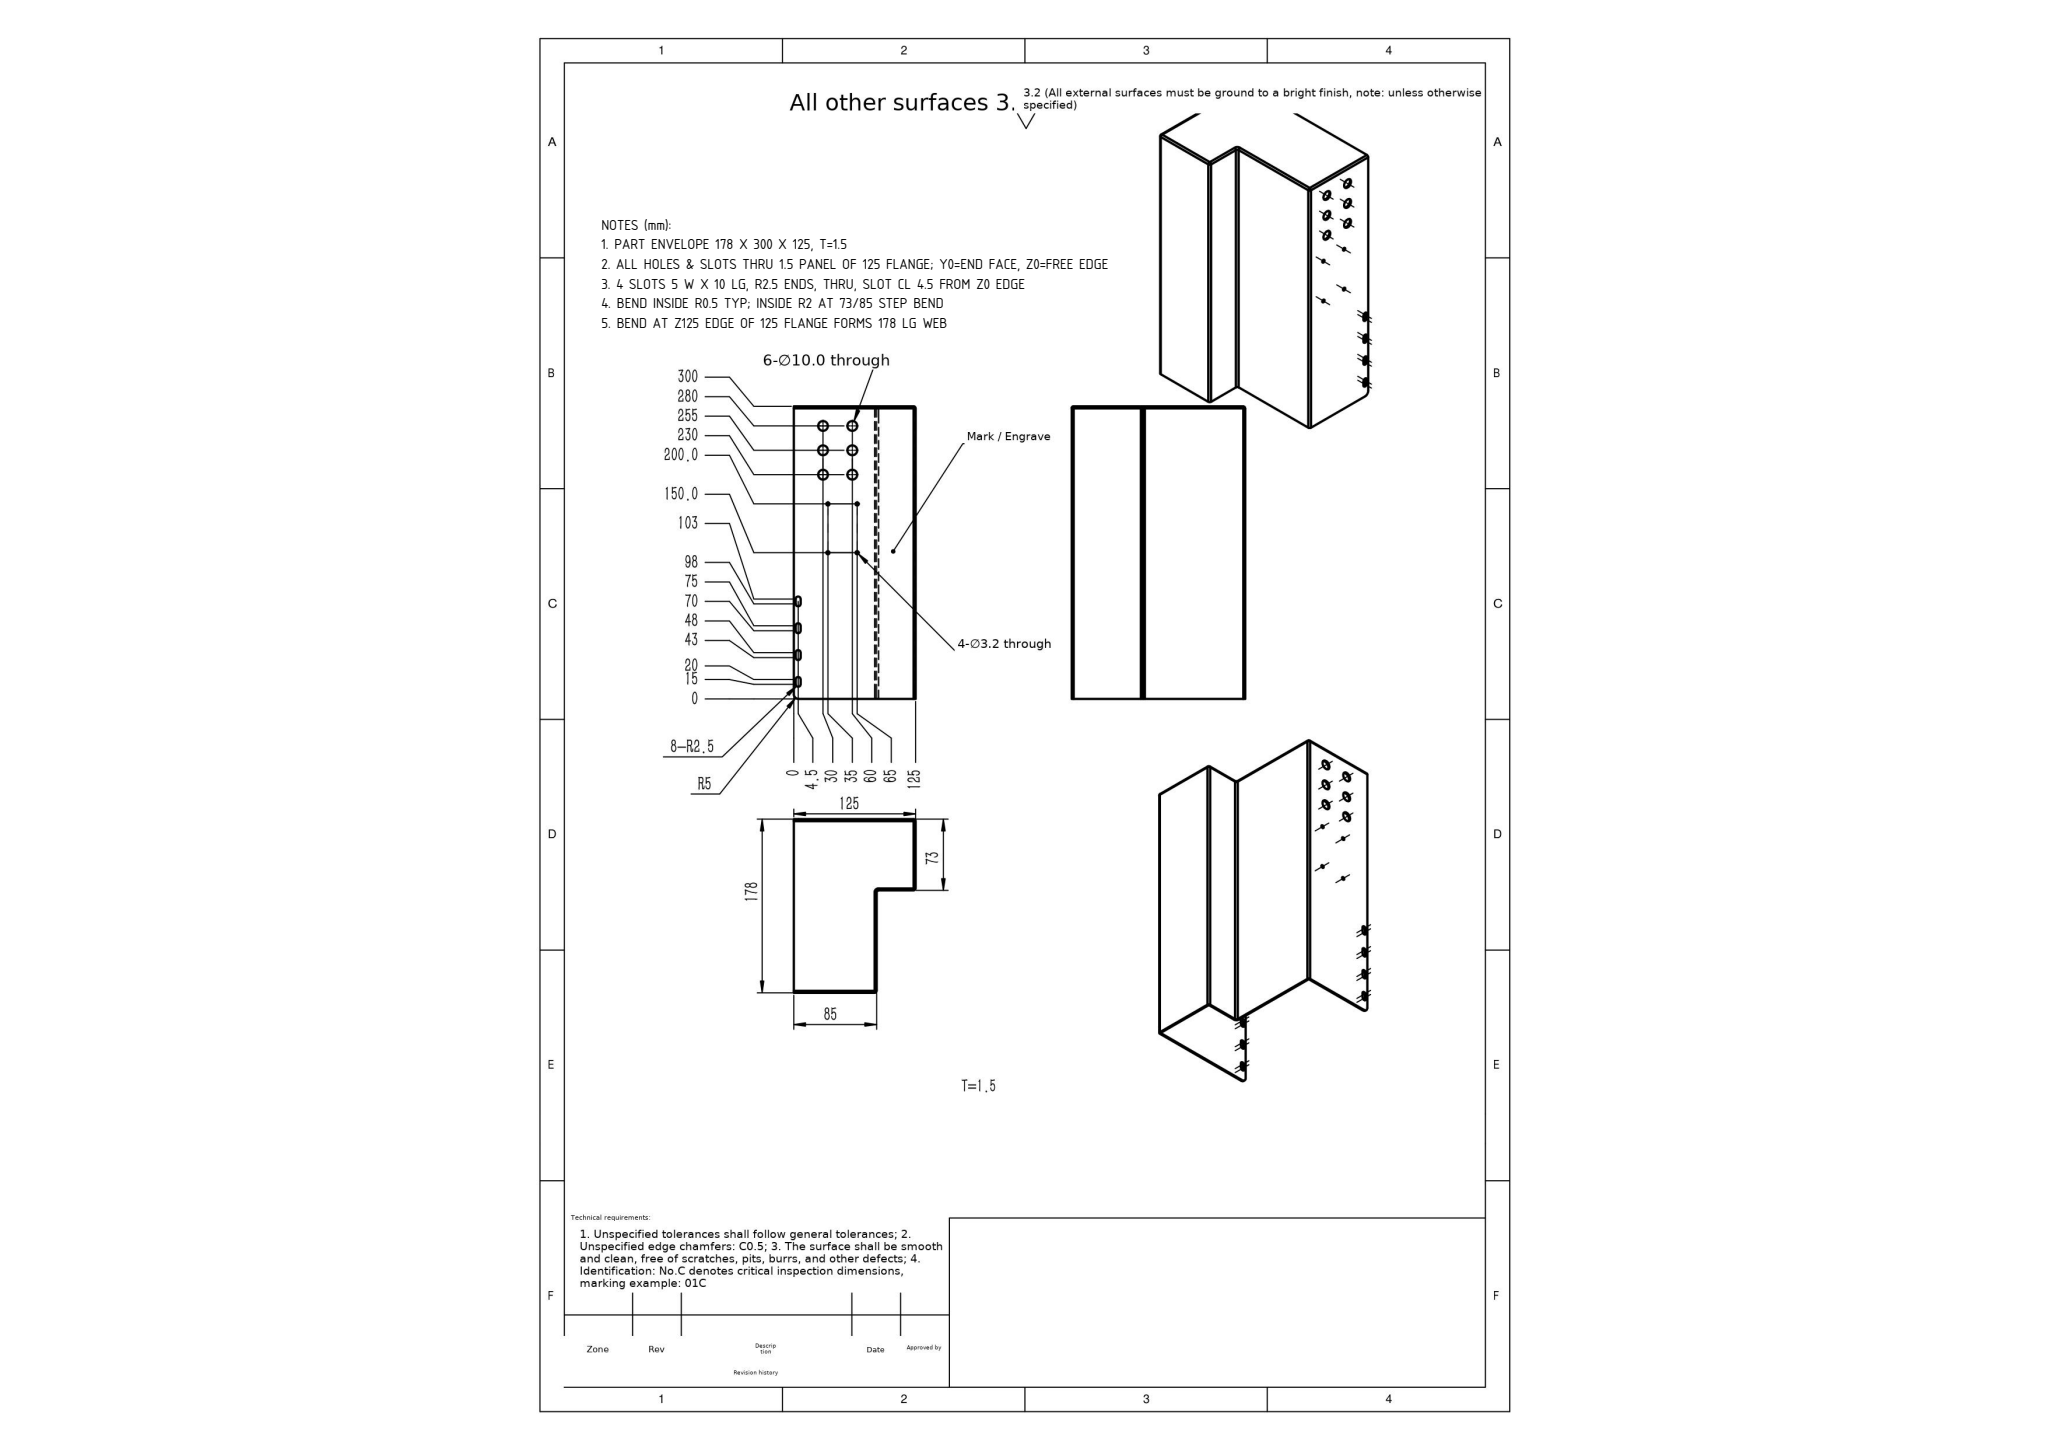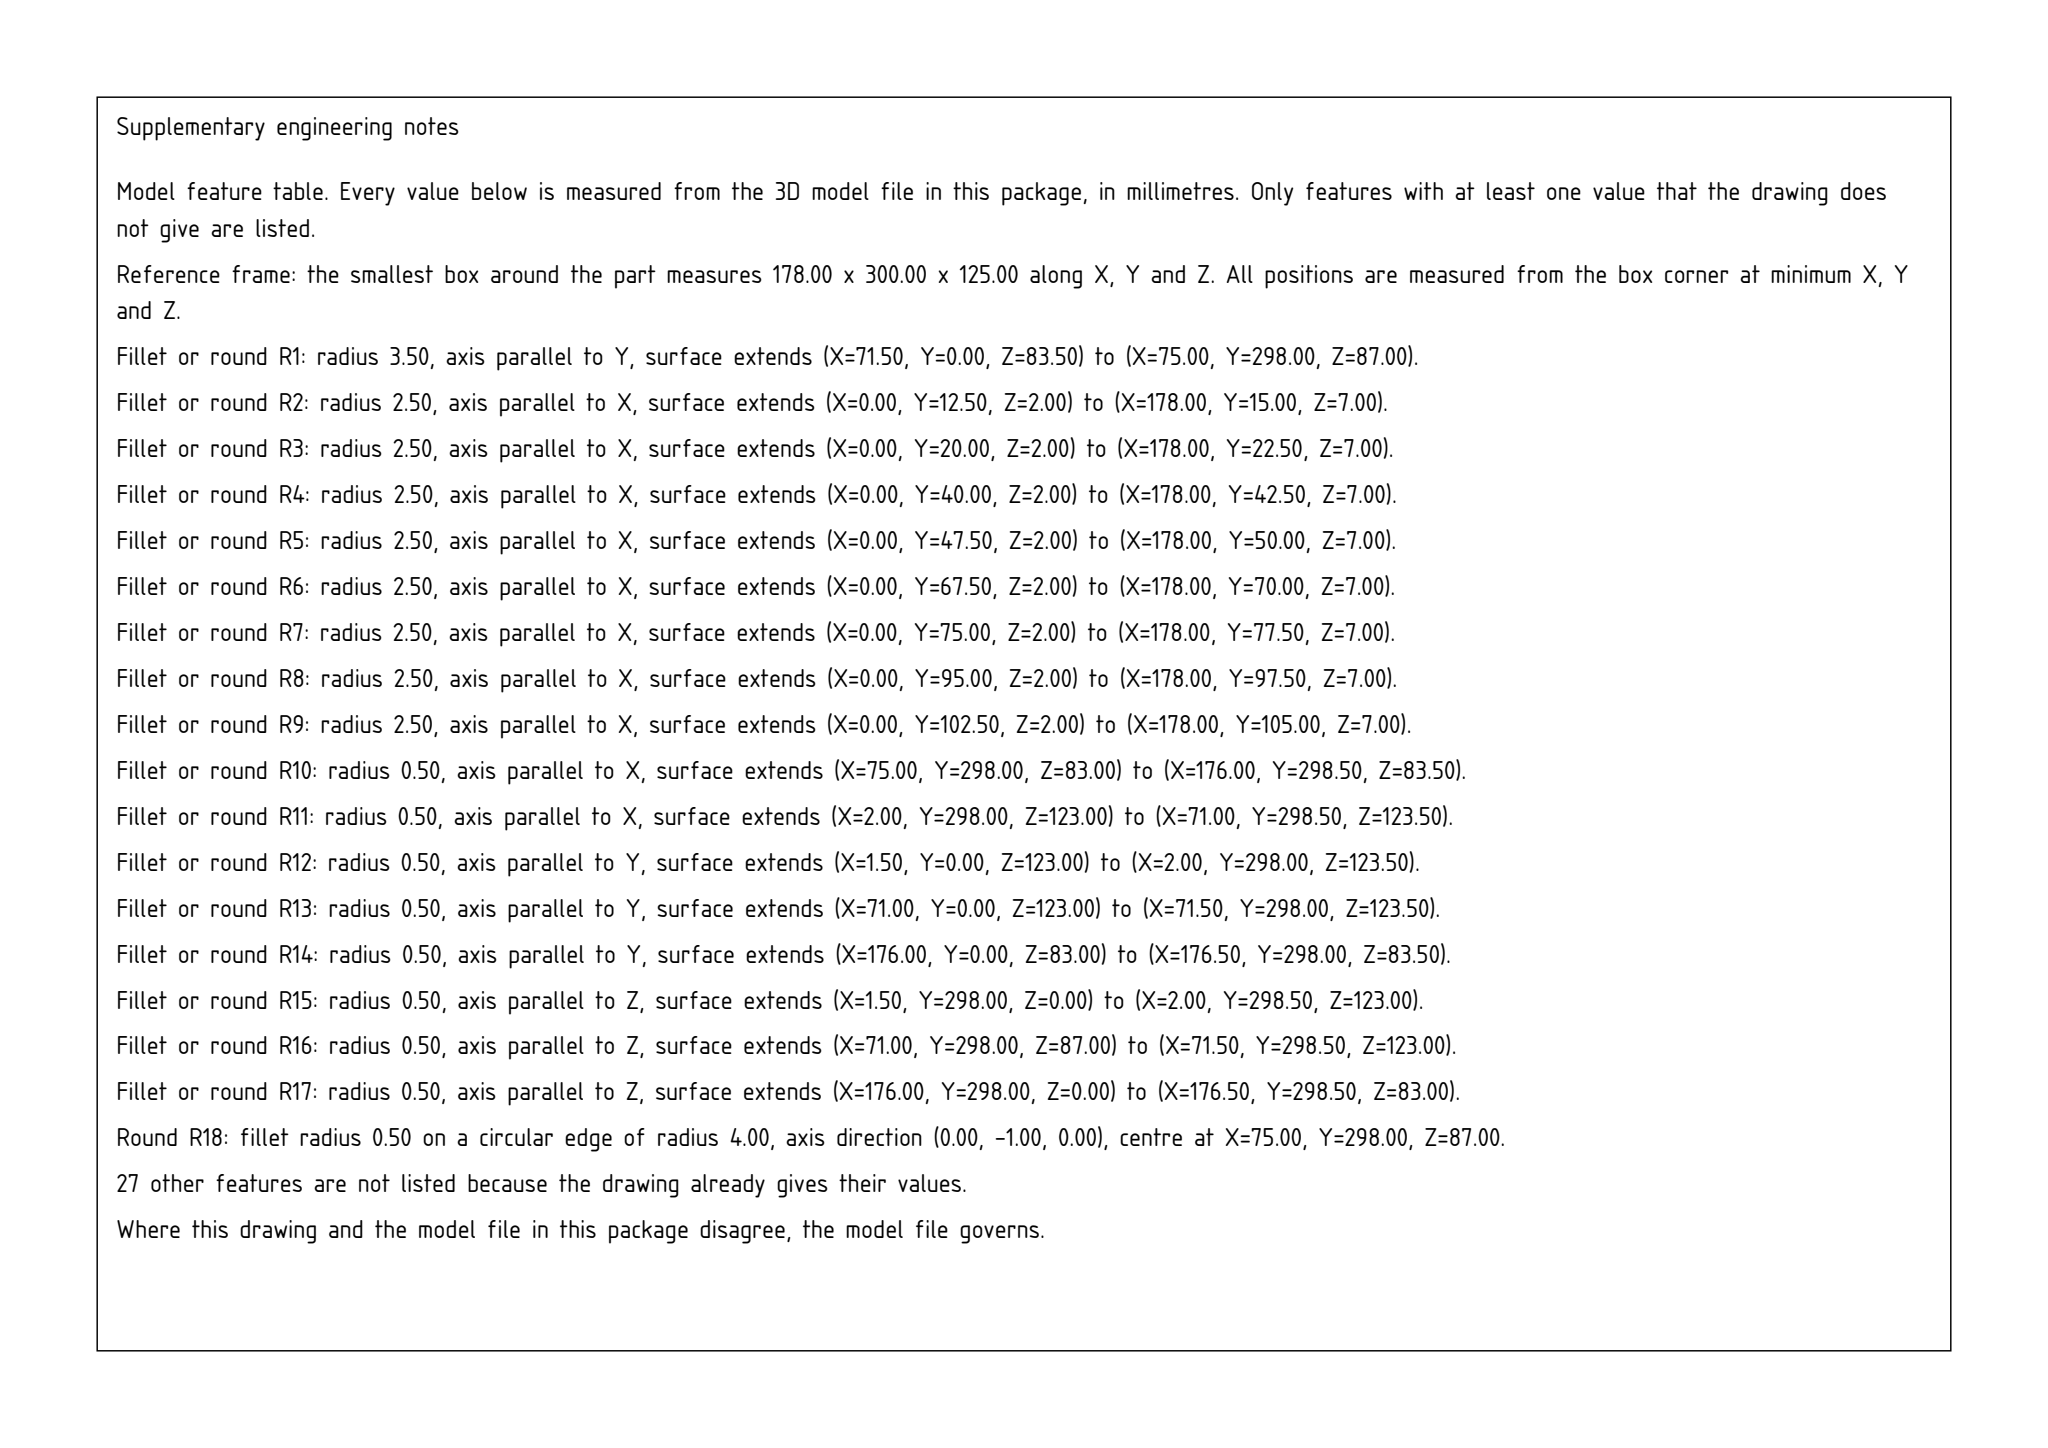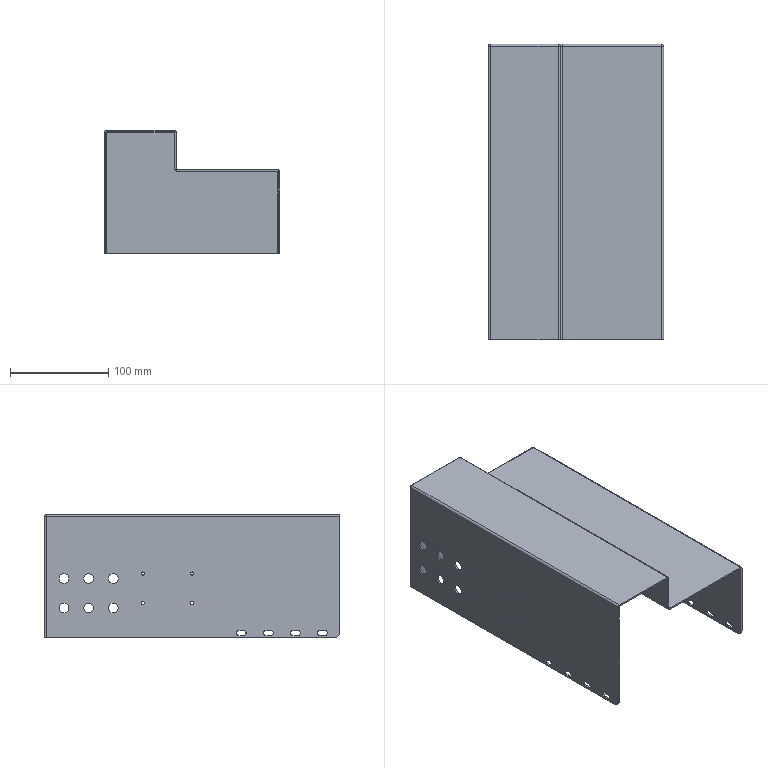Part | SolidWorks | mm | 1 solid | 114 faces | box 178 x 300 x 125 mm | volume 213714 mm3 | cylinder 76 | plane 30 | sphere 6 | torus 2 | commonest cylinder face diameters 10 x26 3.2 x16 5 x16 4 x9 1 x8 7 x1
Drawing notes:
PART ENVELOPE 178 X 300 X 125, T=1.5 | from the solid: bbox_xyz [178,300,125]; paired faces 1.5 apart: x=0/1.5, 71.5/73, 176.5/178
ALL HOLES & SLOTS THRU 1.5 PANEL OF 125 FLANGE; Y0=END FACE, Z0=FREE EDGE | from the solid: Ø3.2, Ø10 and Ø5 slot ends all axis x, len 1.5, in panel x=0-1.5 spanning z=0-125, y=0-300
4 SLOTS 5 W X 10 LG, R2.5 ENDS, THRU, SLOT CL 4.5 FROM Z0 EDGE | from the solid: Ø5 x-axis pairs at z=4.5, y=15/20, 42.5/47.5, 70/75, 97.5/102.5; slot sides z=2.0 & z=7.0 (8 each); 5 ctr-ctr + 5 dia = 10 lg
BEND INSIDE R0.5 TYP; INSIDE R2 AT 73/85 STEP BEND | from the solid: y-axis Ø1/Ø4 at (2,123),(71,123),(176,83) = R0.5 in / R2 out; Ø4/Ø7 at (75,87) = R2 in / R3.5 out; fillet_radii 0.5 & 2.0
BEND AT Z125 EDGE OF 125 FLANGE FORMS 178 LG WEB | from the solid: bend ctr (x=2,z=123) joins panel x=0-1.5 to web z=123.5-125 running x=0-178
build123d program:
from build123d import *

# Parameters (mm, degrees)
SKETCH1_W            = 178
SKETCH1_H            = 300
BOSS_EXTRUDE1_DEPTH  = 125
SKETCH3_W            = 40
SKETCH3_H            = 300
CUT_EXTRUDE2_DEPTH   = 105
FILLET1_R            = 2
SHELL1_T             = -1.5
CUT_EXTRUDE1_DEPTH   = 265.214
LPATTERN1_COUNT      = 4
LPATTERN1_PITCH      = 27.5
SKETCH4_R            = 5
CUT_EXTRUDE3_DEPTH   = 265.214
LPATTERN2_COUNT      = 3
LPATTERN2_PITCH      = 25
SKETCH5_R            = 1.6
CUT_EXTRUDE4_DEPTH   = 265.214
LPATTERN3_COUNT      = 2
LPATTERN3_PITCH      = 30
LPATTERN3_COUNT_DIR2 = 2
LPATTERN3_PITCH_DIR2 = 50
FILLET2_R            = 5


with BuildPart() as part:
    # Sketch1 → Boss-Extrude1 (new body)
    with BuildSketch(Plane.XY):
        Rectangle(SKETCH1_W, SKETCH1_H)
    extrude(amount=BOSS_EXTRUDE1_DEPTH)

    # Sketch3 → Cut-Extrude2 (cut)
    with BuildSketch(Plane(origin=(89, 0, 0), x_dir=(0, 0, -1), z_dir=(1, 0, 0))):
        with Locations((-105, 0)):
            Rectangle(SKETCH3_W, SKETCH3_H)
    extrude(amount=-CUT_EXTRUDE2_DEPTH, mode=Mode.SUBTRACT)

    # Fillet1
    fillet1_edges = [part.edges().sort_by_distance(p)[0] for p in [
        (-89, 0, 125),
        (-52.5, 150, 125),
        (89, 150, 42.5),
        (-16, 0, 125),
        (-16, 150, 105),
        (-16, 0, 85),
        (36.5, 150, 85),
        (89, 0, 85),
        (-89, 150, 62.5),
    ]]
    fillet(fillet1_edges, radius=FILLET1_R)

    # Shell1
    shell1_openings = [part.faces().sort_by_distance(p)[0] for p in [
        (0, -0.004808, 0),
        (-8.494, -150, 52.604),
    ]]
    offset(amount=SHELL1_T, openings=shell1_openings, kind=Kind.INTERSECTION)

    # Sketch2 → Cut-Extrude1 (cut, through all)
    with BuildSketch(Plane(origin=(89, 0, 0), x_dir=(0, 0, -1), z_dir=(1, 0, 0))):
        with BuildLine():
            Line((-2, -130), (-2, -135))
            ThreePointArc((-2, -135), (-4.5, -137.5), (-7, -135))
            Line((-7, -135), (-7, -130))
            ThreePointArc((-7, -130), (-4.5, -127.5), (-2, -130))
        make_face()
    cut_extrude1 = extrude(amount=-CUT_EXTRUDE1_DEPTH, mode=Mode.SUBTRACT)

    # LPattern1: Cut-Extrude1 ×4
    with Locations(*[(0, i * LPATTERN1_PITCH, 0) for i in range(1, LPATTERN1_COUNT)]):
        add(cut_extrude1, mode=Mode.SUBTRACT)

    # Sketch4 → Cut-Extrude3 (cut, through all)
    with BuildSketch(Plane(origin=(89, 0, 0), x_dir=(0, 0, -1), z_dir=(1, 0, 0))):
        with Locations((-60, 130)):
            Circle(SKETCH4_R)
        with Locations((-30, 130)):
            Circle(SKETCH4_R)
    cut_extrude3 = extrude(amount=-CUT_EXTRUDE3_DEPTH, mode=Mode.SUBTRACT)

    # LPattern2: Cut-Extrude3 ×3
    with Locations(*[(0, -i * LPATTERN2_PITCH, 0) for i in range(1, LPATTERN2_COUNT)]):
        add(cut_extrude3, mode=Mode.SUBTRACT)

    # Sketch5 → Cut-Extrude4 (cut, through all)
    with BuildSketch(Plane(origin=(89, 0, 0), x_dir=(0, 0, -1), z_dir=(1, 0, 0))):
        with Locations((-65, 50)):
            Circle(SKETCH5_R)
    cut_extrude4 = extrude(amount=-CUT_EXTRUDE4_DEPTH, mode=Mode.SUBTRACT)

    # LPattern3: Cut-Extrude4 2 × 2
    with Locations(*[(0, -j * LPATTERN3_PITCH_DIR2, -i * LPATTERN3_PITCH) for i in range(LPATTERN3_COUNT) for j in range(LPATTERN3_COUNT_DIR2) if (i, j) != (0, 0)]):
        add(cut_extrude4, mode=Mode.SUBTRACT)

    # Fillet2
    fillet2_edges = [part.edges().sort_by_distance(p)[0] for p in [
        (-88.25, -150, 0),
        (88.25, -150, 0),
    ]]
    fillet(fillet2_edges, radius=FILLET2_R)


solid = part.part